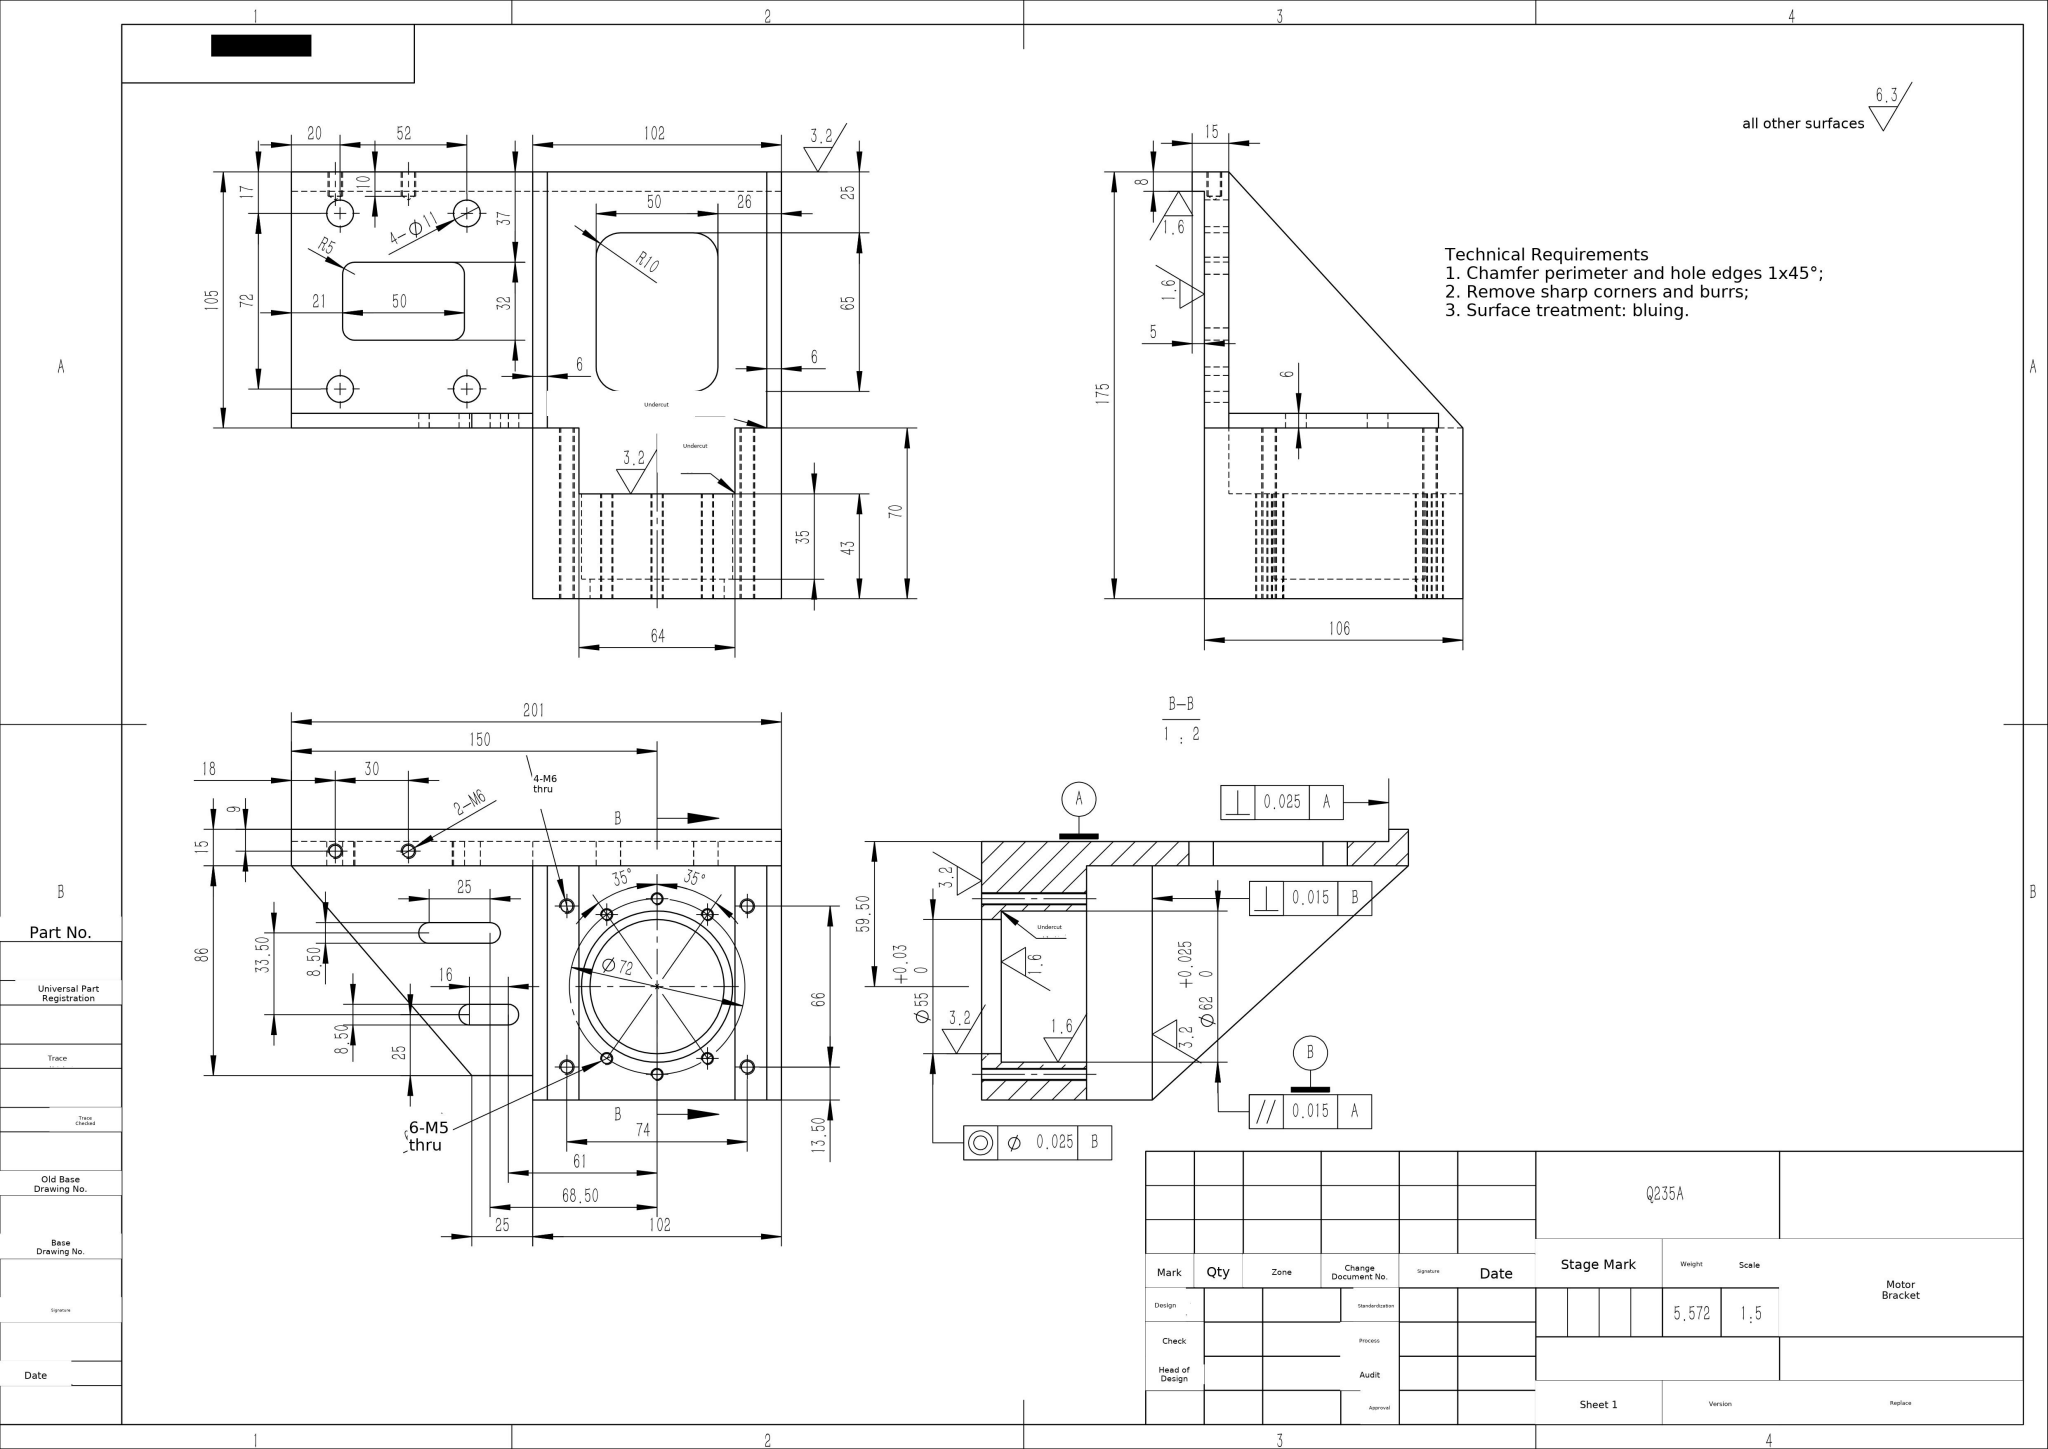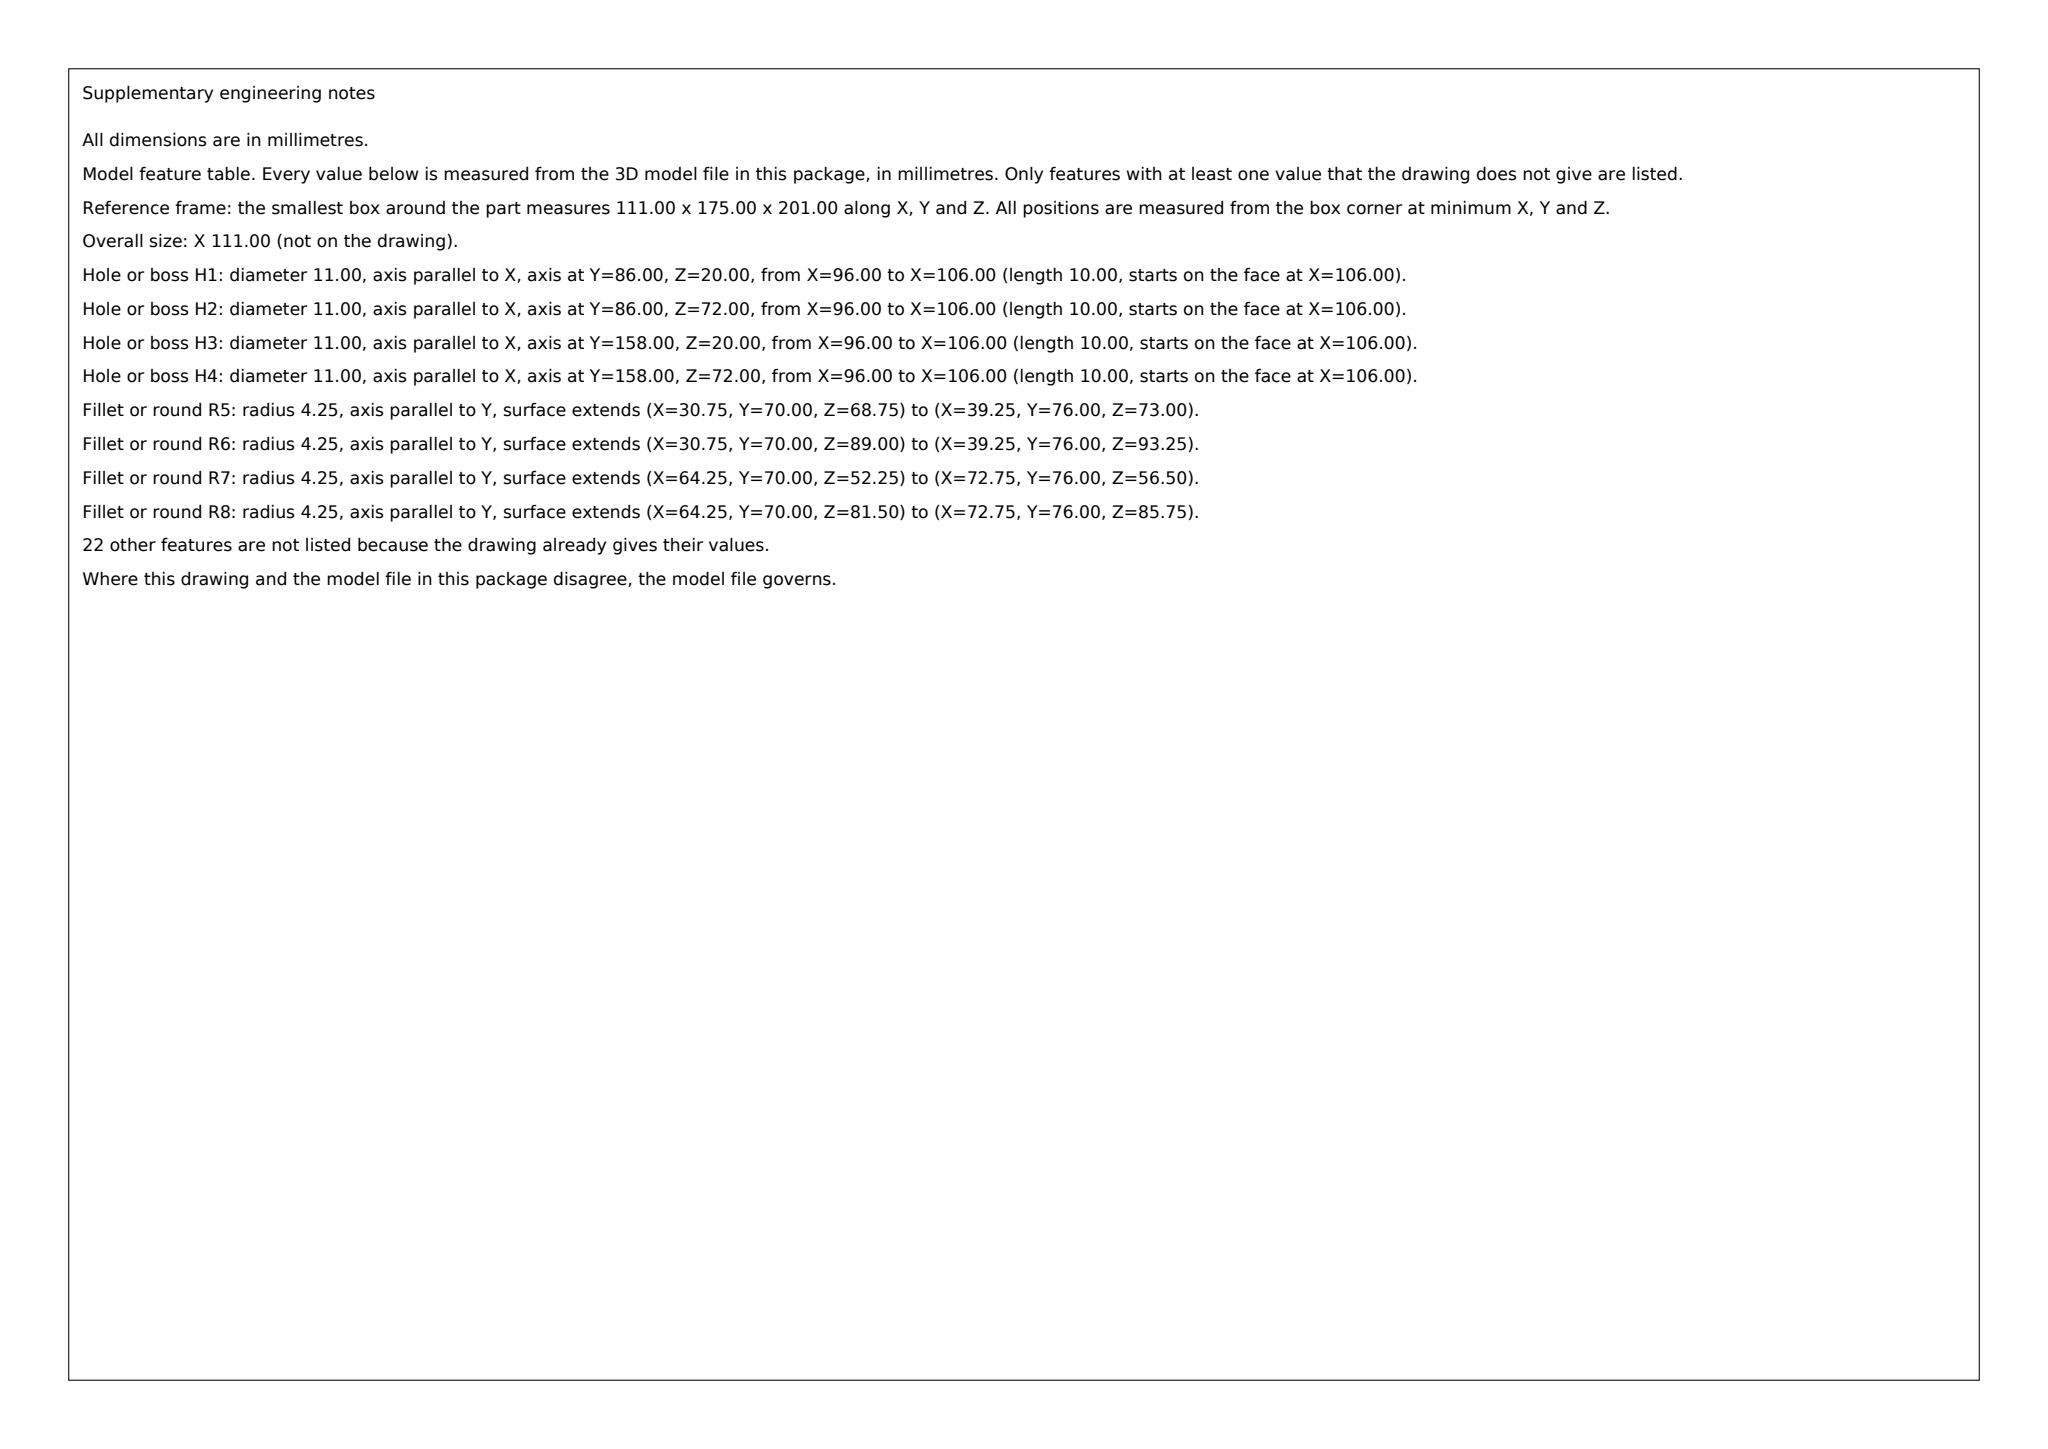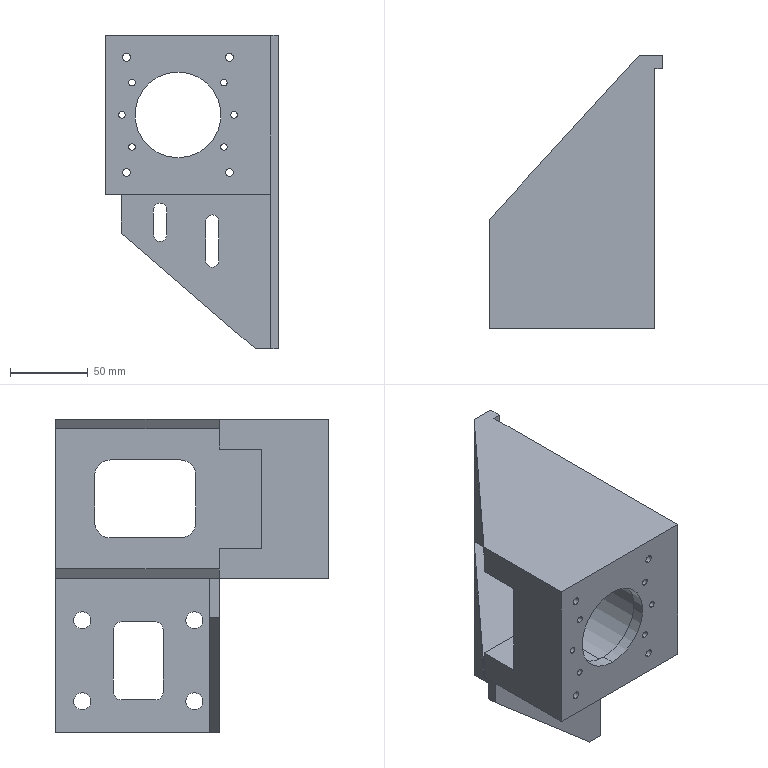Part | SolidWorks | mm | material Q235A | 1 solid | 91 faces | box 111 x 175 x 201 mm | volume 714355 mm3 | cylinder 50 | plane 37 | cone 4 | commonest cylinder face diameters 5 x12 4.2 x12 11 x8 8.5 x6 20 x4 10 x4 62 x2 55 x2
build123d program:
from build123d import *

# Parameters (mm, degrees)
SKETCH1_W             = 104
SKETCH1_H             = 102
BOSS_EXTRUDE1_DEPTH   = 70
SKETCH2_R             = 27.5
CUT_EXTRUDE1_DEPTH    = 8
SKETCH3_R             = 31
CUT_EXTRUDE2_DEPTH    = 35
SKETCH4_W             = 96
SKETCH4_H             = 64
CUT_EXTRUDE3_DEPTH    = 27
SKETCH8_W             = 8
SKETCH8_H             = 102
BOSS_EXTRUDE2_DEPTH   = 105
BOSS_EXTRUDE3_DEPTH   = 6
SKETCH13_W            = 13
SKETCH13_H            = 31
CUT_EXTRUDE6_DEPTH    = 210.124
BOSS_EXTRUDE4_START   = -144
SKETCH14_W            = 18
SKETCH14_H            = 201
BOSS_EXTRUDE4_DEPTH   = 144
BOSS_EXTRUDE5_DEPTH   = 6
SKETCH17_R            = 5.5
CUT_EXTRUDE8_DEPTH    = 250.682
CUT_EXTRUDE10_DEPTH   = 20
CUT_EXTRUDE11_DEPTH   = 250.682
SKETCH21_W            = 99
SKETCH21_H            = 39
CUT_EXTRUDE12_DEPTH   = 250.682
SKETCH23_W            = 102
SKETCH23_H            = 31
BOSS_EXTRUDE6_DEPTH   = 23
CUT_EXTRUDE14_START   = -201
SKETCH24_W            = 8
SKETCH24_H            = 167
CUT_EXTRUDE14_DEPTH   = 201
CUT_EXTRUDE15_START   = -201
SKETCH26_W            = 3
SKETCH26_H            = 8
CUT_EXTRUDE15_DEPTH   = 201
M6_TAPPED_HOLE1_D     = 5
M5_TAPPED_HOLE1_D     = 4.2
M6_TAPPED_HOLE2_D     = 5
M6_TAPPED_HOLE2_DEPTH = 10
M6_TAPPED_HOLE2_TIP   = 1.502
CUT_EXTRUDE16_DEPTH   = 10


with BuildPart() as part:
    # Sketch1 → Boss-Extrude1 (new body)
    with BuildSketch(Plane(origin=(0, 0, 0), x_dir=(1, 0, 0), z_dir=(0, 1, 0))):
        Rectangle(SKETCH1_W, SKETCH1_H)
    extrude(amount=BOSS_EXTRUDE1_DEPTH)

    # Sketch2 → Cut-Extrude1 (cut)
    with BuildSketch(Plane.XZ):
        with Locations(Location((-5.5, 0, 0), (0, 0, 270))):
            Circle(SKETCH2_R)
    extrude(amount=-CUT_EXTRUDE1_DEPTH, mode=Mode.SUBTRACT)

    # Sketch3 → Cut-Extrude2 (cut)
    with BuildSketch(Plane.XZ.offset(-8)):
        with Locations(Location((-5.5, 0, 0), (0, 0, 270))):
            Circle(SKETCH3_R)
    extrude(amount=-CUT_EXTRUDE2_DEPTH, mode=Mode.SUBTRACT)

    # Sketch4 → Cut-Extrude3 (cut)
    with BuildSketch(Plane(origin=(0, 70, 0), x_dir=(1, 0, 0), z_dir=(0, 1, 0))):
        with Locations((-4, 0)):
            Rectangle(SKETCH4_W, SKETCH4_H)
    extrude(amount=-CUT_EXTRUDE3_DEPTH, mode=Mode.SUBTRACT)

    # Sketch8 → Boss-Extrude2 (add)
    with BuildSketch(Plane(origin=(0, 70, 0), x_dir=(1, 0, 0), z_dir=(0, 1, 0))):
        with Locations((48, 0)):
            Rectangle(SKETCH8_W, SKETCH8_H)
    extrude(amount=BOSS_EXTRUDE2_DEPTH)

    # Sketch9 → Boss-Extrude3 (add)
    with BuildSketch(Plane.XY.offset(51)):
        Polygon((-52, 70), (44, 175), (44, 70), align=None)
    boss_extrude3 = extrude(amount=-BOSS_EXTRUDE3_DEPTH)

    # Mirror1: Boss-Extrude3 across plane
    add(boss_extrude3.mirror(Plane.XY))

    # Sketch13 → Cut-Extrude6 (cut, through all)
    with BuildSketch(Plane.XY.offset(51)):
        with Locations((45.5, 15.5)):
            Rectangle(SKETCH13_W, SKETCH13_H)
    extrude(amount=-CUT_EXTRUDE6_DEPTH, mode=Mode.SUBTRACT)

    # Sketch14 → Boss-Extrude4 (add)
    with BuildSketch(Plane(origin=(0, 175, 0), x_dir=(1, 0, 0), z_dir=(0, 1, 0)).offset(BOSS_EXTRUDE4_START)):
        with Locations((53, 49.5)):
            Rectangle(SKETCH14_W, SKETCH14_H)
    extrude(amount=BOSS_EXTRUDE4_DEPTH)

    # Sketch15 → Boss-Extrude5 (add)
    with BuildSketch(Plane(origin=(0, 70, 0), x_dir=(-1, 0, 0), z_dir=(0, -1, 0))):
        Polygon((42, 51), (42, 76), (-44, 150), (-44, 51), align=None)
    extrude(amount=-BOSS_EXTRUDE5_DEPTH)

    # Sketch17 → Cut-Extrude8 (cut, through all)
    with BuildSketch(Plane.ZY.offset(-44)):
        with Locations((-130, 158)):
            Circle(SKETCH17_R)
        with Locations((-78, 158)):
            Circle(SKETCH17_R)
        with Locations((-130, 86)):
            Circle(SKETCH17_R)
        with Locations((-78, 86)):
            Circle(SKETCH17_R)
    extrude(amount=-CUT_EXTRUDE8_DEPTH, mode=Mode.SUBTRACT)

    # Sketch19 → Cut-Extrude10 (cut)
    with BuildSketch(Plane.ZY.offset(-44)):
        with BuildLine():
            Line((-15, 150), (15, 150))
            ThreePointArc((15, 150), (22.071, 147.071), (25, 140))
            Line((25, 140), (25, 95))
            ThreePointArc((25, 95), (22.071, 87.929), (15, 85))
            Line((15, 85), (-15, 85))
            ThreePointArc((-15, 85), (-22.071, 87.929), (-25, 95))
            Line((-25, 95), (-25, 140))
            ThreePointArc((-25, 140), (-22.071, 147.071), (-15, 150))
        make_face()
    extrude(amount=-CUT_EXTRUDE10_DEPTH, mode=Mode.SUBTRACT)

    # Sketch20 → Cut-Extrude11 (cut, through all)
    with BuildSketch(Plane.ZY.offset(-44)):
        with BuildLine():
            Line((-124, 138), (-84, 138))
            ThreePointArc((-84, 138), (-80.464, 136.536), (-79, 133))
            Line((-79, 133), (-79, 111))
            ThreePointArc((-79, 111), (-80.464, 107.464), (-84, 106))
            Line((-84, 106), (-124, 106))
            ThreePointArc((-124, 106), (-127.536, 107.464), (-129, 111))
            Line((-129, 111), (-129, 133))
            ThreePointArc((-129, 133), (-127.536, 136.536), (-124, 138))
        make_face()
    extrude(amount=-CUT_EXTRUDE11_DEPTH, mode=Mode.SUBTRACT)

    # Sketch21 → Cut-Extrude12 (cut, through all)
    with BuildSketch(Plane.ZY.offset(-44)):
        with Locations((-100.5, 50.5)):
            Rectangle(SKETCH21_W, SKETCH21_H)
    extrude(amount=-CUT_EXTRUDE12_DEPTH, mode=Mode.SUBTRACT)

    # Sketch23 → Boss-Extrude6 (add)
    with BuildSketch(Plane(origin=(39, 0, 0), x_dir=(0, 0, -1), z_dir=(1, 0, 0))):
        with Locations((0, 15.5)):
            Rectangle(SKETCH23_W, SKETCH23_H)
    extrude(amount=BOSS_EXTRUDE6_DEPTH)

    # Sketch24 → Cut-Extrude14 (cut)
    with BuildSketch(Plane(origin=(0, 0, -150), x_dir=(-1, 0, 0), z_dir=(0, 0, -1)).offset(CUT_EXTRUDE14_START)):
        with Locations((-58, 83.5)):
            Rectangle(SKETCH24_W, SKETCH24_H)
    extrude(amount=CUT_EXTRUDE14_DEPTH, mode=Mode.SUBTRACT)

    # Sketch26 → Cut-Extrude15 (cut)
    with BuildSketch(Plane.XY.offset(51).offset(CUT_EXTRUDE15_START)):
        with Locations((60.5, 171)):
            Rectangle(SKETCH26_W, SKETCH26_H)
    extrude(amount=CUT_EXTRUDE15_DEPTH, mode=Mode.SUBTRACT)

    # M6 Tapped Hole1 (through all)
    with Locations(Plane(origin=(0, 70, 0), x_dir=(1, 0, 0), z_dir=(0, 1, 0))):
        with Locations((-38.5, 37), (27.5, 37), (-38.5, -37), (27.5, -37)):
            Hole(M6_TAPPED_HOLE1_D / 2)

    # M5 Tapped Hole1 (through all)
    with Locations(Plane(origin=(0, 43, 0), x_dir=(1, 0, 0), z_dir=(0, 1, 0))):
        with Locations((-34.989, 20.649), (-41.5, 0), (-34.989, -20.649), (23.989, -20.649), (30.5, 0), (23.989, 20.649)):
            Hole(M5_TAPPED_HOLE1_D / 2)

    # M6 Tapped Hole2
    with Locations(Plane(origin=(0, 175, 0), x_dir=(1, 0, 0), z_dir=(0, 1, 0))):
        with Locations((50, 132), (50, 102)):
            Hole(M6_TAPPED_HOLE2_D / 2, depth=M6_TAPPED_HOLE2_DEPTH)
            with Locations((0, 0, -(M6_TAPPED_HOLE2_DEPTH + M6_TAPPED_HOLE2_TIP / 2))):  # 118° drill point
                Cone(0, M6_TAPPED_HOLE2_D / 2, M6_TAPPED_HOLE2_TIP, mode=Mode.SUBTRACT)

    # Sketch34 → Cut-Extrude16 (cut)
    with BuildSketch(Plane(origin=(0, 76, 0), x_dir=(1, 0, 0), z_dir=(0, 1, 0))):
        with BuildLine():
            Line((20.75, 93.5), (20.75, 68.5))
            ThreePointArc((20.75, 68.5), (16.5, 64.25), (12.25, 68.5))
            Line((12.25, 68.5), (12.25, 93.5))
            ThreePointArc((12.25, 93.5), (16.5, 97.75), (20.75, 93.5))
        make_face()
        with BuildLine():
            Line((-12.75, 77), (-12.75, 61))
            ThreePointArc((-12.75, 61), (-17, 56.75), (-21.25, 61))
            Line((-21.25, 61), (-21.25, 77))
            ThreePointArc((-21.25, 77), (-17, 81.25), (-12.75, 77))
        make_face()
    extrude(amount=-CUT_EXTRUDE16_DEPTH, mode=Mode.SUBTRACT)


solid = part.part